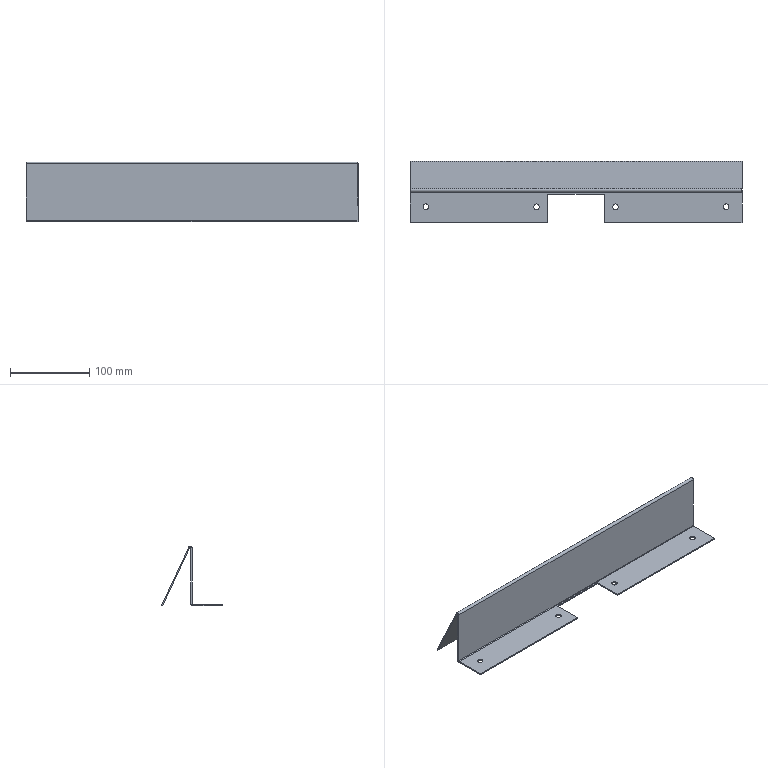Component | SolidWorks | Q1-A12-S21-Q4-05B-1 | 1 solid | 34 faces | box 420 x 77.3 x 75.36 mm | volume 119609 mm3 | plane 22 | cylinder 12 | commonest cylinder face diameters 7 x8 4.473 x2 1.473 x2 | material SUS-304
STEP:
#1=COLOUR_RGB('',0.7922,0.8196,0.9333);
#2=FILL_AREA_STYLE_COLOUR('',#1);
#3=FILL_AREA_STYLE('',(#2));
#4=SURFACE_STYLE_FILL_AREA(#3);
#5=SURFACE_SIDE_STYLE('',(#4));
#6=SURFACE_STYLE_USAGE(.BOTH.,#5);
#7=PRESENTATION_STYLE_ASSIGNMENT((#6));
#8=CARTESIAN_POINT('',(31.181,-0.7874,5.906));
#9=VERTEX_POINT('',#8);
#10=CARTESIAN_POINT('',(30.906,-0.7874,5.906));
#11=VERTEX_POINT('',#10);
#12=CARTESIAN_POINT('',(31.043,-0.7874,5.906));
#13=DIRECTION('',(0.,0.,-1.));
#14=DIRECTION('',(-1.,0.,0.));
#15=AXIS2_PLACEMENT_3D('',#12,#13,#14);
#16=CIRCLE('',#15,0.1378);
#17=EDGE_CURVE('',#9,#11,#16,.T.);
#18=ORIENTED_EDGE('',*,*,#17,.T.);
#19=CARTESIAN_POINT('',(30.906,-0.7874,5.965));
#20=VERTEX_POINT('',#19);
#21=CARTESIAN_POINT('',(30.906,-0.7874,5.965));
#22=DIRECTION('',(0.,0.,1.));
#23=VECTOR('',#22,39.37);
#24=LINE('',#21,#23);
#25=EDGE_CURVE('',#11,#20,#24,.T.);
#26=ORIENTED_EDGE('',*,*,#25,.T.);
#27=CARTESIAN_POINT('',(31.181,-0.7874,5.965));
#28=VERTEX_POINT('',#27);
#29=CARTESIAN_POINT('',(31.043,-0.7874,5.965));
#30=DIRECTION('',(0.,0.,1.));
#31=DIRECTION('',(1.,0.,0.));
#32=AXIS2_PLACEMENT_3D('',#29,#30,#31);
#33=CIRCLE('',#32,0.1378);
#34=EDGE_CURVE('',#20,#28,#33,.T.);
#35=ORIENTED_EDGE('',*,*,#34,.T.);
#36=CARTESIAN_POINT('',(31.181,-0.7874,5.965));
#37=DIRECTION('',(0.,0.,1.));
#38=VECTOR('',#37,39.37);
#39=LINE('',#36,#38);
#40=EDGE_CURVE('',#9,#28,#39,.T.);
#41=ORIENTED_EDGE('',*,*,#40,.F.);
#42=EDGE_LOOP('',(#18,#26,#35,#41));
#43=FACE_OUTER_BOUND('',#42,.T.);
#44=CARTESIAN_POINT('',(31.043,-0.7874,5.965));
#45=DIRECTION('',(0.,0.,1.));
#46=DIRECTION('',(1.,0.,0.));
#47=AXIS2_PLACEMENT_3D('',#44,#45,#46);
#48=CYLINDRICAL_SURFACE('',#47,0.1378);
#49=ADVANCED_FACE('',(#43),#48,.F.);
#50=CARTESIAN_POINT('',(25.669,-0.7874,5.906));
#51=VERTEX_POINT('',#50);
#52=CARTESIAN_POINT('',(25.394,-0.7874,5.906));
#53=VERTEX_POINT('',#52);
#54=CARTESIAN_POINT('',(25.531,-0.7874,5.906));
#55=DIRECTION('',(0.,0.,-1.));
#56=DIRECTION('',(-1.,0.,0.));
#57=AXIS2_PLACEMENT_3D('',#54,#55,#56);
#58=CIRCLE('',#57,0.1378);
#59=EDGE_CURVE('',#51,#53,#58,.T.);
#60=ORIENTED_EDGE('',*,*,#59,.T.);
#61=CARTESIAN_POINT('',(25.394,-0.7874,5.965));
#62=VERTEX_POINT('',#61);
#63=CARTESIAN_POINT('',(25.394,-0.7874,5.965));
#64=DIRECTION('',(0.,0.,1.));
#65=VECTOR('',#64,39.37);
#66=LINE('',#63,#65);
#67=EDGE_CURVE('',#53,#62,#66,.T.);
#68=ORIENTED_EDGE('',*,*,#67,.T.);
#69=CARTESIAN_POINT('',(25.669,-0.7874,5.965));
#70=VERTEX_POINT('',#69);
#71=CARTESIAN_POINT('',(25.531,-0.7874,5.965));
#72=DIRECTION('',(0.,0.,1.));
#73=DIRECTION('',(1.,0.,0.));
#74=AXIS2_PLACEMENT_3D('',#71,#72,#73);
#75=CIRCLE('',#74,0.1378);
#76=EDGE_CURVE('',#62,#70,#75,.T.);
#77=ORIENTED_EDGE('',*,*,#76,.T.);
#78=CARTESIAN_POINT('',(25.669,-0.7874,5.965));
#79=DIRECTION('',(0.,0.,1.));
#80=VECTOR('',#79,39.37);
#81=LINE('',#78,#80);
#82=EDGE_CURVE('',#51,#70,#81,.T.);
#83=ORIENTED_EDGE('',*,*,#82,.F.);
#84=EDGE_LOOP('',(#60,#68,#77,#83));
#85=FACE_OUTER_BOUND('',#84,.T.);
#86=CARTESIAN_POINT('',(25.531,-0.7874,5.965));
#87=DIRECTION('',(0.,0.,1.));
#88=DIRECTION('',(1.,0.,0.));
#89=AXIS2_PLACEMENT_3D('',#86,#87,#88);
#90=CYLINDRICAL_SURFACE('',#89,0.1378);
#91=ADVANCED_FACE('',(#85),#90,.F.);
#92=CARTESIAN_POINT('',(21.732,-0.7874,5.906));
#93=VERTEX_POINT('',#92);
#94=CARTESIAN_POINT('',(21.457,-0.7874,5.906));
#95=VERTEX_POINT('',#94);
#96=CARTESIAN_POINT('',(21.594,-0.7874,5.906));
#97=DIRECTION('',(0.,0.,-1.));
#98=DIRECTION('',(-1.,0.,0.));
#99=AXIS2_PLACEMENT_3D('',#96,#97,#98);
#100=CIRCLE('',#99,0.1378);
#101=EDGE_CURVE('',#93,#95,#100,.T.);
#102=ORIENTED_EDGE('',*,*,#101,.T.);
#103=CARTESIAN_POINT('',(21.457,-0.7874,5.965));
#104=VERTEX_POINT('',#103);
#105=CARTESIAN_POINT('',(21.457,-0.7874,5.965));
#106=DIRECTION('',(0.,0.,1.));
#107=VECTOR('',#106,39.37);
#108=LINE('',#105,#107);
#109=EDGE_CURVE('',#95,#104,#108,.T.);
#110=ORIENTED_EDGE('',*,*,#109,.T.);
#111=CARTESIAN_POINT('',(21.732,-0.7874,5.965));
#112=VERTEX_POINT('',#111);
#113=CARTESIAN_POINT('',(21.594,-0.7874,5.965));
#114=DIRECTION('',(0.,0.,1.));
#115=DIRECTION('',(1.,0.,0.));
#116=AXIS2_PLACEMENT_3D('',#113,#114,#115);
#117=CIRCLE('',#116,0.1378);
#118=EDGE_CURVE('',#104,#112,#117,.T.);
#119=ORIENTED_EDGE('',*,*,#118,.T.);
#120=CARTESIAN_POINT('',(21.732,-0.7874,5.965));
#121=DIRECTION('',(0.,0.,1.));
#122=VECTOR('',#121,39.37);
#123=LINE('',#120,#122);
#124=EDGE_CURVE('',#93,#112,#123,.T.);
#125=ORIENTED_EDGE('',*,*,#124,.F.);
#126=EDGE_LOOP('',(#102,#110,#119,#125));
#127=FACE_OUTER_BOUND('',#126,.T.);
#128=CARTESIAN_POINT('',(21.594,-0.7874,5.965));
#129=DIRECTION('',(0.,0.,1.));
#130=DIRECTION('',(1.,0.,0.));
#131=AXIS2_PLACEMENT_3D('',#128,#129,#130);
#132=CYLINDRICAL_SURFACE('',#131,0.1378);
#133=ADVANCED_FACE('',(#127),#132,.F.);
#134=CARTESIAN_POINT('',(16.22,-0.7874,5.906));
#135=VERTEX_POINT('',#134);
#136=CARTESIAN_POINT('',(15.945,-0.7874,5.906));
#137=VERTEX_POINT('',#136);
#138=CARTESIAN_POINT('',(16.083,-0.7874,5.906));
#139=DIRECTION('',(0.,0.,-1.));
#140=DIRECTION('',(-1.,0.,0.));
#141=AXIS2_PLACEMENT_3D('',#138,#139,#140);
#142=CIRCLE('',#141,0.1378);
#143=EDGE_CURVE('',#135,#137,#142,.T.);
#144=ORIENTED_EDGE('',*,*,#143,.T.);
#145=CARTESIAN_POINT('',(15.945,-0.7874,5.965));
#146=VERTEX_POINT('',#145);
#147=CARTESIAN_POINT('',(15.945,-0.7874,5.965));
#148=DIRECTION('',(0.,0.,1.));
#149=VECTOR('',#148,39.37);
#150=LINE('',#147,#149);
#151=EDGE_CURVE('',#137,#146,#150,.T.);
#152=ORIENTED_EDGE('',*,*,#151,.T.);
#153=CARTESIAN_POINT('',(16.22,-0.7874,5.965));
#154=VERTEX_POINT('',#153);
#155=CARTESIAN_POINT('',(16.083,-0.7874,5.965));
#156=DIRECTION('',(0.,0.,1.));
#157=DIRECTION('',(1.,0.,0.));
#158=AXIS2_PLACEMENT_3D('',#155,#156,#157);
#159=CIRCLE('',#158,0.1378);
#160=EDGE_CURVE('',#146,#154,#159,.T.);
#161=ORIENTED_EDGE('',*,*,#160,.T.);
#162=CARTESIAN_POINT('',(16.22,-0.7874,5.965));
#163=DIRECTION('',(0.,0.,1.));
#164=VECTOR('',#163,39.37);
#165=LINE('',#162,#164);
#166=EDGE_CURVE('',#135,#154,#165,.T.);
#167=ORIENTED_EDGE('',*,*,#166,.F.);
#168=EDGE_LOOP('',(#144,#152,#161,#167));
#169=FACE_OUTER_BOUND('',#168,.T.);
#170=CARTESIAN_POINT('',(16.083,-0.7874,5.965));
#171=DIRECTION('',(0.,0.,1.));
#172=DIRECTION('',(1.,0.,0.));
#173=AXIS2_PLACEMENT_3D('',#170,#171,#172);
#174=CYLINDRICAL_SURFACE('',#173,0.1378);
#175=ADVANCED_FACE('',(#169),#174,.F.);
#176=CARTESIAN_POINT('',(31.831,0.05528,8.797));
#177=VERTEX_POINT('',#176);
#178=CARTESIAN_POINT('',(31.831,1.404,5.906));
#179=VERTEX_POINT('',#178);
#180=CARTESIAN_POINT('',(31.831,1.518,5.66));
#181=DIRECTION('',(0.,0.4226,-0.9063));
#182=VECTOR('',#181,39.37);
#183=LINE('',#180,#182);
#184=EDGE_CURVE('',#177,#179,#183,.T.);
#185=ORIENTED_EDGE('',*,*,#184,.T.);
#186=CARTESIAN_POINT('',(31.831,1.469,5.906));
#187=VERTEX_POINT('',#186);
#188=CARTESIAN_POINT('',(31.831,1.572,5.906));
#189=DIRECTION('',(0.,1.,0.));
#190=VECTOR('',#189,39.37);
#191=LINE('',#188,#190);
#192=EDGE_CURVE('',#179,#187,#191,.T.);
#193=ORIENTED_EDGE('',*,*,#192,.T.);
#194=CARTESIAN_POINT('',(31.831,0.1088,8.822));
#195=VERTEX_POINT('',#194);
#196=CARTESIAN_POINT('',(31.831,1.097,6.703));
#197=DIRECTION('',(0.,0.4226,-0.9063));
#198=VECTOR('',#197,39.37);
#199=LINE('',#196,#198);
#200=EDGE_CURVE('',#195,#187,#199,.T.);
#201=ORIENTED_EDGE('',*,*,#200,.F.);
#202=CARTESIAN_POINT('',(31.831,0.05528,8.797));
#203=DIRECTION('',(0.,0.9063,0.4226));
#204=VECTOR('',#203,39.37);
#205=LINE('',#202,#204);
#206=EDGE_CURVE('',#177,#195,#205,.T.);
#207=ORIENTED_EDGE('',*,*,#206,.F.);
#208=EDGE_LOOP('',(#185,#193,#201,#207));
#209=FACE_OUTER_BOUND('',#208,.T.);
#210=CARTESIAN_POINT('',(31.831,1.572,5.685));
#211=DIRECTION('',(-1.,0.,0.));
#212=DIRECTION('',(0.,0.,1.));
#213=AXIS2_PLACEMENT_3D('',#210,#211,#212);
#214=PLANE('',#213);
#215=ADVANCED_FACE('',(#209),#214,.F.);
#216=CARTESIAN_POINT('',(15.295,1.469,5.906));
#217=VERTEX_POINT('',#216);
#218=CARTESIAN_POINT('',(15.295,0.1088,8.822));
#219=VERTEX_POINT('',#218);
#220=CARTESIAN_POINT('',(15.295,1.097,6.703));
#221=DIRECTION('',(0.,-0.4226,0.9063));
#222=VECTOR('',#221,39.37);
#223=LINE('',#220,#222);
#224=EDGE_CURVE('',#217,#219,#223,.T.);
#225=ORIENTED_EDGE('',*,*,#224,.F.);
#226=CARTESIAN_POINT('',(15.295,1.404,5.906));
#227=VERTEX_POINT('',#226);
#228=CARTESIAN_POINT('',(15.295,0.05352,5.906));
#229=DIRECTION('',(0.,-1.,0.));
#230=VECTOR('',#229,39.37);
#231=LINE('',#228,#230);
#232=EDGE_CURVE('',#217,#227,#231,.T.);
#233=ORIENTED_EDGE('',*,*,#232,.T.);
#234=CARTESIAN_POINT('',(15.295,0.05528,8.797));
#235=VERTEX_POINT('',#234);
#236=CARTESIAN_POINT('',(15.295,0.,8.915));
#237=DIRECTION('',(0.,-0.4226,0.9063));
#238=VECTOR('',#237,39.37);
#239=LINE('',#236,#238);
#240=EDGE_CURVE('',#227,#235,#239,.T.);
#241=ORIENTED_EDGE('',*,*,#240,.T.);
#242=CARTESIAN_POINT('',(15.295,0.1088,8.822));
#243=DIRECTION('',(0.,0.9063,0.4226));
#244=VECTOR('',#243,39.37);
#245=LINE('',#242,#244);
#246=EDGE_CURVE('',#235,#219,#245,.T.);
#247=ORIENTED_EDGE('',*,*,#246,.T.);
#248=EDGE_LOOP('',(#225,#233,#241,#247));
#249=FACE_OUTER_BOUND('',#248,.T.);
#250=CARTESIAN_POINT('',(15.295,0.05352,8.94));
#251=DIRECTION('',(1.,0.,0.));
#252=DIRECTION('',(0.,0.,-1.));
#253=AXIS2_PLACEMENT_3D('',#250,#251,#252);
#254=PLANE('',#253);
#255=ADVANCED_FACE('',(#249),#254,.F.);
#256=ORIENTED_EDGE('',*,*,#200,.T.);
#257=CARTESIAN_POINT('',(23.563,1.469,5.906));
#258=DIRECTION('',(-1.,0.,0.));
#259=VECTOR('',#258,39.37);
#260=LINE('',#257,#259);
#261=EDGE_CURVE('',#187,#217,#260,.T.);
#262=ORIENTED_EDGE('',*,*,#261,.T.);
#263=ORIENTED_EDGE('',*,*,#224,.T.);
#264=CARTESIAN_POINT('',(15.295,0.1088,8.822));
#265=DIRECTION('',(-1.,0.,-0.));
#266=VECTOR('',#265,39.37);
#267=LINE('',#264,#266);
#268=EDGE_CURVE('',#195,#219,#267,.T.);
#269=ORIENTED_EDGE('',*,*,#268,.F.);
#270=EDGE_LOOP('',(#256,#262,#263,#269));
#271=FACE_OUTER_BOUND('',#270,.T.);
#272=CARTESIAN_POINT('',(23.563,1.097,6.703));
#273=DIRECTION('',(0.,-0.9063,-0.4226));
#274=DIRECTION('',(0.,0.4226,-0.9063));
#275=AXIS2_PLACEMENT_3D('',#272,#273,#274);
#276=PLANE('',#275);
#277=ADVANCED_FACE('',(#271),#276,.F.);
#278=CARTESIAN_POINT('',(23.563,1.404,5.906));
#279=DIRECTION('',(-1.,0.,0.));
#280=VECTOR('',#279,39.37);
#281=LINE('',#278,#280);
#282=EDGE_CURVE('',#179,#227,#281,.T.);
#283=ORIENTED_EDGE('',*,*,#282,.F.);
#284=ORIENTED_EDGE('',*,*,#184,.F.);
#285=CARTESIAN_POINT('',(15.295,0.05528,8.797));
#286=DIRECTION('',(1.,-0.,0.));
#287=VECTOR('',#286,39.37);
#288=LINE('',#285,#287);
#289=EDGE_CURVE('',#235,#177,#288,.T.);
#290=ORIENTED_EDGE('',*,*,#289,.F.);
#291=ORIENTED_EDGE('',*,*,#240,.F.);
#292=EDGE_LOOP('',(#283,#284,#290,#291));
#293=FACE_OUTER_BOUND('',#292,.T.);
#294=CARTESIAN_POINT('',(23.563,1.043,6.678));
#295=DIRECTION('',(0.,-0.9063,-0.4226));
#296=DIRECTION('',(0.,0.4226,-0.9063));
#297=AXIS2_PLACEMENT_3D('',#294,#295,#296);
#298=PLANE('',#297);
#299=ADVANCED_FACE('',(#293),#298,.T.);
#300=CARTESIAN_POINT('',(22.146,-1.575,5.965));
#301=VERTEX_POINT('',#300);
#302=CARTESIAN_POINT('',(22.146,-1.575,5.906));
#303=VERTEX_POINT('',#302);
#304=CARTESIAN_POINT('',(22.146,-1.575,5.906));
#305=DIRECTION('',(0.,0.,-1.));
#306=VECTOR('',#305,39.37);
#307=LINE('',#304,#306);
#308=EDGE_CURVE('',#301,#303,#307,.T.);
#309=ORIENTED_EDGE('',*,*,#308,.F.);
#310=CARTESIAN_POINT('',(15.295,-1.575,5.965));
#311=VERTEX_POINT('',#310);
#312=CARTESIAN_POINT('',(15.295,-1.575,5.965));
#313=DIRECTION('',(1.,0.,0.));
#314=VECTOR('',#313,39.37);
#315=LINE('',#312,#314);
#316=EDGE_CURVE('',#311,#301,#315,.T.);
#317=ORIENTED_EDGE('',*,*,#316,.F.);
#318=CARTESIAN_POINT('',(15.295,-1.575,5.906));
#319=VERTEX_POINT('',#318);
#320=CARTESIAN_POINT('',(15.295,-1.575,5.906));
#321=DIRECTION('',(0.,0.,1.));
#322=VECTOR('',#321,39.37);
#323=LINE('',#320,#322);
#324=EDGE_CURVE('',#319,#311,#323,.T.);
#325=ORIENTED_EDGE('',*,*,#324,.F.);
#326=CARTESIAN_POINT('',(15.295,-1.575,5.906));
#327=DIRECTION('',(1.,0.,0.));
#328=VECTOR('',#327,39.37);
#329=LINE('',#326,#328);
#330=EDGE_CURVE('',#319,#303,#329,.T.);
#331=ORIENTED_EDGE('',*,*,#330,.T.);
#332=EDGE_LOOP('',(#309,#317,#325,#331));
#333=FACE_OUTER_BOUND('',#332,.T.);
#334=CARTESIAN_POINT('',(15.295,-1.575,5.906));
#335=DIRECTION('',(0.,-1.,0.));
#336=DIRECTION('',(0.,0.,-1.));
#337=AXIS2_PLACEMENT_3D('',#334,#335,#336);
#338=PLANE('',#337);
#339=ADVANCED_FACE('',(#333),#338,.T.);
#340=CARTESIAN_POINT('',(15.295,0.,8.785));
#341=VERTEX_POINT('',#340);
#342=CARTESIAN_POINT('',(15.295,-0.05906,8.785));
#343=VERTEX_POINT('',#342);
#344=CARTESIAN_POINT('',(15.295,0.,8.785));
#345=DIRECTION('',(0.,-1.,0.));
#346=VECTOR('',#345,39.37);
#347=LINE('',#344,#346);
#348=EDGE_CURVE('',#341,#343,#347,.T.);
#349=ORIENTED_EDGE('',*,*,#348,.F.);
#350=CARTESIAN_POINT('',(15.295,-0.,5.994));
#351=VERTEX_POINT('',#350);
#352=CARTESIAN_POINT('',(15.295,-0.,5.965));
#353=DIRECTION('',(-0.,0.,1.));
#354=VECTOR('',#353,39.37);
#355=LINE('',#352,#354);
#356=EDGE_CURVE('',#351,#341,#355,.T.);
#357=ORIENTED_EDGE('',*,*,#356,.F.);
#358=CARTESIAN_POINT('',(15.295,-0.05906,5.994));
#359=VERTEX_POINT('',#358);
#360=CARTESIAN_POINT('',(15.295,-0.05906,5.994));
#361=DIRECTION('',(0.,1.,-0.));
#362=VECTOR('',#361,39.37);
#363=LINE('',#360,#362);
#364=EDGE_CURVE('',#359,#351,#363,.T.);
#365=ORIENTED_EDGE('',*,*,#364,.F.);
#366=CARTESIAN_POINT('',(15.295,-0.05906,9.055));
#367=DIRECTION('',(-0.,0.,1.));
#368=VECTOR('',#367,39.37);
#369=LINE('',#366,#368);
#370=EDGE_CURVE('',#359,#343,#369,.T.);
#371=ORIENTED_EDGE('',*,*,#370,.T.);
#372=EDGE_LOOP('',(#349,#357,#365,#371));
#373=FACE_OUTER_BOUND('',#372,.T.);
#374=CARTESIAN_POINT('',(15.295,0.,9.055));
#375=DIRECTION('',(1.,0.,0.));
#376=DIRECTION('',(0.,0.,-1.));
#377=AXIS2_PLACEMENT_3D('',#374,#375,#376);
#378=PLANE('',#377);
#379=ADVANCED_FACE('',(#373),#378,.F.);
#380=CARTESIAN_POINT('',(31.831,0.,8.785));
#381=VERTEX_POINT('',#380);
#382=CARTESIAN_POINT('',(31.831,-0.05906,8.785));
#383=VERTEX_POINT('',#382);
#384=CARTESIAN_POINT('',(31.831,0.,8.785));
#385=DIRECTION('',(0.,-1.,0.));
#386=VECTOR('',#385,39.37);
#387=LINE('',#384,#386);
#388=EDGE_CURVE('',#381,#383,#387,.T.);
#389=ORIENTED_EDGE('',*,*,#388,.T.);
#390=CARTESIAN_POINT('',(31.831,-0.05906,5.994));
#391=VERTEX_POINT('',#390);
#392=CARTESIAN_POINT('',(31.831,-0.05906,5.965));
#393=DIRECTION('',(0.,-0.,-1.));
#394=VECTOR('',#393,39.37);
#395=LINE('',#392,#394);
#396=EDGE_CURVE('',#383,#391,#395,.T.);
#397=ORIENTED_EDGE('',*,*,#396,.T.);
#398=CARTESIAN_POINT('',(31.831,-0.,5.994));
#399=VERTEX_POINT('',#398);
#400=CARTESIAN_POINT('',(31.831,-0.,5.994));
#401=DIRECTION('',(0.,1.,-0.));
#402=VECTOR('',#401,39.37);
#403=LINE('',#400,#402);
#404=EDGE_CURVE('',#391,#399,#403,.T.);
#405=ORIENTED_EDGE('',*,*,#404,.T.);
#406=CARTESIAN_POINT('',(31.831,-0.,5.965));
#407=DIRECTION('',(0.,-0.,-1.));
#408=VECTOR('',#407,39.37);
#409=LINE('',#406,#408);
#410=EDGE_CURVE('',#381,#399,#409,.T.);
#411=ORIENTED_EDGE('',*,*,#410,.F.);
#412=EDGE_LOOP('',(#389,#397,#405,#411));
#413=FACE_OUTER_BOUND('',#412,.T.);
#414=CARTESIAN_POINT('',(31.831,-0.,5.965));
#415=DIRECTION('',(-1.,-0.,-0.));
#416=DIRECTION('',(-0.,0.,1.));
#417=AXIS2_PLACEMENT_3D('',#414,#415,#416);
#418=PLANE('',#417);
#419=ADVANCED_FACE('',(#413),#418,.F.);
#420=CARTESIAN_POINT('',(31.831,0.,8.785));
#421=DIRECTION('',(-1.,0.,0.));
#422=VECTOR('',#421,39.37);
#423=LINE('',#420,#422);
#424=EDGE_CURVE('',#381,#341,#423,.T.);
#425=ORIENTED_EDGE('',*,*,#424,.F.);
#426=ORIENTED_EDGE('',*,*,#410,.T.);
#427=CARTESIAN_POINT('',(31.831,-0.,5.994));
#428=DIRECTION('',(1.,-0.,-0.));
#429=VECTOR('',#428,39.37);
#430=LINE('',#427,#429);
#431=EDGE_CURVE('',#351,#399,#430,.T.);
#432=ORIENTED_EDGE('',*,*,#431,.F.);
#433=ORIENTED_EDGE('',*,*,#356,.T.);
#434=EDGE_LOOP('',(#425,#426,#432,#433));
#435=FACE_OUTER_BOUND('',#434,.T.);
#436=CARTESIAN_POINT('',(23.563,-0.,5.965));
#437=DIRECTION('',(0.,-1.,0.));
#438=DIRECTION('',(0.,-0.,-1.));
#439=AXIS2_PLACEMENT_3D('',#436,#437,#438);
#440=PLANE('',#439);
#441=ADVANCED_FACE('',(#435),#440,.F.);
#442=ORIENTED_EDGE('',*,*,#396,.F.);
#443=CARTESIAN_POINT('',(31.831,-0.05906,8.785));
#444=DIRECTION('',(-1.,0.,0.));
#445=VECTOR('',#444,39.37);
#446=LINE('',#443,#445);
#447=EDGE_CURVE('',#383,#343,#446,.T.);
#448=ORIENTED_EDGE('',*,*,#447,.T.);
#449=ORIENTED_EDGE('',*,*,#370,.F.);
#450=CARTESIAN_POINT('',(31.831,-0.05906,5.994));
#451=DIRECTION('',(-1.,0.,0.));
#452=VECTOR('',#451,39.37);
#453=LINE('',#450,#452);
#454=EDGE_CURVE('',#391,#359,#453,.T.);
#455=ORIENTED_EDGE('',*,*,#454,.F.);
#456=EDGE_LOOP('',(#442,#448,#449,#455));
#457=FACE_OUTER_BOUND('',#456,.T.);
#458=CARTESIAN_POINT('',(23.563,-0.05906,5.965));
#459=DIRECTION('',(0.,-1.,0.));
#460=DIRECTION('',(0.,-0.,-1.));
#461=AXIS2_PLACEMENT_3D('',#458,#459,#460);
#462=PLANE('',#461);
#463=ADVANCED_FACE('',(#457),#462,.T.);
#464=CARTESIAN_POINT('',(15.295,-0.08806,5.965));
#465=VERTEX_POINT('',#464);
#466=CARTESIAN_POINT('',(15.295,-1.575,5.965));
#467=DIRECTION('',(0.,-1.,0.));
#468=VECTOR('',#467,39.37);
#469=LINE('',#466,#468);
#470=EDGE_CURVE('',#465,#311,#469,.T.);
#471=ORIENTED_EDGE('',*,*,#470,.F.);
#472=CARTESIAN_POINT('',(15.295,-0.08806,5.906));
#473=VERTEX_POINT('',#472);
#474=CARTESIAN_POINT('',(15.295,-0.08806,5.965));
#475=DIRECTION('',(0.,0.,-1.));
#476=VECTOR('',#475,39.37);
#477=LINE('',#474,#476);
#478=EDGE_CURVE('',#465,#473,#477,.T.);
#479=ORIENTED_EDGE('',*,*,#478,.T.);
#480=CARTESIAN_POINT('',(15.295,-1.575,5.906));
#481=DIRECTION('',(0.,-1.,0.));
#482=VECTOR('',#481,39.37);
#483=LINE('',#480,#482);
#484=EDGE_CURVE('',#473,#319,#483,.T.);
#485=ORIENTED_EDGE('',*,*,#484,.T.);
#486=ORIENTED_EDGE('',*,*,#324,.T.);
#487=EDGE_LOOP('',(#471,#479,#485,#486));
#488=FACE_OUTER_BOUND('',#487,.T.);
#489=CARTESIAN_POINT('',(15.295,-1.575,5.906));
#490=DIRECTION('',(-1.,0.,0.));
#491=DIRECTION('',(0.,0.,1.));
#492=AXIS2_PLACEMENT_3D('',#489,#490,#491);
#493=PLANE('',#492);
#494=ADVANCED_FACE('',(#488),#493,.T.);
#495=ORIENTED_EDGE('',*,*,#17,.F.);
#496=CARTESIAN_POINT('',(31.043,-0.7874,5.906));
#497=DIRECTION('',(0.,0.,-1.));
#498=DIRECTION('',(-1.,0.,0.));
#499=AXIS2_PLACEMENT_3D('',#496,#497,#498);
#500=CIRCLE('',#499,0.1378);
#501=EDGE_CURVE('',#11,#9,#500,.T.);
#502=ORIENTED_EDGE('',*,*,#501,.F.);
#503=EDGE_LOOP('',(#495,#502));
#504=FACE_BOUND('',#503,.T.);
#505=ORIENTED_EDGE('',*,*,#59,.F.);
#506=CARTESIAN_POINT('',(25.531,-0.7874,5.906));
#507=DIRECTION('',(0.,0.,-1.));
#508=DIRECTION('',(-1.,0.,0.));
#509=AXIS2_PLACEMENT_3D('',#506,#507,#508);
#510=CIRCLE('',#509,0.1378);
#511=EDGE_CURVE('',#53,#51,#510,.T.);
#512=ORIENTED_EDGE('',*,*,#511,.F.);
#513=EDGE_LOOP('',(#505,#512));
#514=FACE_BOUND('',#513,.T.);
#515=ORIENTED_EDGE('',*,*,#101,.F.);
#516=CARTESIAN_POINT('',(21.594,-0.7874,5.906));
#517=DIRECTION('',(0.,0.,-1.));
#518=DIRECTION('',(-1.,0.,0.));
#519=AXIS2_PLACEMENT_3D('',#516,#517,#518);
#520=CIRCLE('',#519,0.1378);
#521=EDGE_CURVE('',#95,#93,#520,.T.);
#522=ORIENTED_EDGE('',*,*,#521,.F.);
#523=EDGE_LOOP('',(#515,#522));
#524=FACE_BOUND('',#523,.T.);
#525=ORIENTED_EDGE('',*,*,#143,.F.);
#526=CARTESIAN_POINT('',(16.083,-0.7874,5.906));
#527=DIRECTION('',(0.,0.,-1.));
#528=DIRECTION('',(-1.,0.,0.));
#529=AXIS2_PLACEMENT_3D('',#526,#527,#528);
#530=CIRCLE('',#529,0.1378);
#531=EDGE_CURVE('',#137,#135,#530,.T.);
#532=ORIENTED_EDGE('',*,*,#531,.F.);
#533=EDGE_LOOP('',(#525,#532));
#534=FACE_BOUND('',#533,.T.);
#535=CARTESIAN_POINT('',(22.146,-0.1575,5.906));
#536=VERTEX_POINT('',#535);
#537=CARTESIAN_POINT('',(22.146,-0.7874,5.906));
#538=DIRECTION('',(0.,1.,0.));
#539=VECTOR('',#538,39.37);
#540=LINE('',#537,#539);
#541=EDGE_CURVE('',#303,#536,#540,.T.);
#542=ORIENTED_EDGE('',*,*,#541,.F.);
#543=ORIENTED_EDGE('',*,*,#330,.F.);
#544=ORIENTED_EDGE('',*,*,#484,.F.);
#545=CARTESIAN_POINT('',(31.831,-0.08806,5.906));
#546=VERTEX_POINT('',#545);
#547=CARTESIAN_POINT('',(15.295,-0.08806,5.906));
#548=DIRECTION('',(1.,0.,0.));
#549=VECTOR('',#548,39.37);
#550=LINE('',#547,#549);
#551=EDGE_CURVE('',#473,#546,#550,.T.);
#552=ORIENTED_EDGE('',*,*,#551,.T.);
#553=CARTESIAN_POINT('',(31.831,-1.575,5.906));
#554=VERTEX_POINT('',#553);
#555=CARTESIAN_POINT('',(31.831,-1.575,5.906));
#556=DIRECTION('',(0.,1.,0.));
#557=VECTOR('',#556,39.37);
#558=LINE('',#555,#557);
#559=EDGE_CURVE('',#554,#546,#558,.T.);
#560=ORIENTED_EDGE('',*,*,#559,.F.);
#561=CARTESIAN_POINT('',(24.98,-1.575,5.906));
#562=VERTEX_POINT('',#561);
#563=CARTESIAN_POINT('',(15.295,-1.575,5.906));
#564=DIRECTION('',(1.,0.,0.));
#565=VECTOR('',#564,39.37);
#566=LINE('',#563,#565);
#567=EDGE_CURVE('',#562,#554,#566,.T.);
#568=ORIENTED_EDGE('',*,*,#567,.F.);
#569=CARTESIAN_POINT('',(24.98,-0.1575,5.906));
#570=VERTEX_POINT('',#569);
#571=CARTESIAN_POINT('',(24.98,-0.7874,5.906));
#572=DIRECTION('',(0.,-1.,0.));
#573=VECTOR('',#572,39.37);
#574=LINE('',#571,#573);
#575=EDGE_CURVE('',#570,#562,#574,.T.);
#576=ORIENTED_EDGE('',*,*,#575,.F.);
#577=CARTESIAN_POINT('',(23.563,-0.1575,5.906));
#578=DIRECTION('',(1.,0.,0.));
#579=VECTOR('',#578,39.37);
#580=LINE('',#577,#579);
#581=EDGE_CURVE('',#536,#570,#580,.T.);
#582=ORIENTED_EDGE('',*,*,#581,.F.);
#583=EDGE_LOOP('',(#542,#543,#544,#552,#560,#568,#576,#582));
#584=FACE_OUTER_BOUND('',#583,.T.);
#585=CARTESIAN_POINT('',(23.563,-0.7874,5.906));
#586=DIRECTION('',(0.,0.,-1.));
#587=DIRECTION('',(-1.,0.,0.));
#588=AXIS2_PLACEMENT_3D('',#585,#586,#587);
#589=PLANE('',#588);
#590=ADVANCED_FACE('',(#504,#514,#524,#534,#584),#589,.T.);
#591=CARTESIAN_POINT('',(31.043,-0.7874,5.965));
#592=DIRECTION('',(0.,0.,1.));
#593=DIRECTION('',(1.,0.,0.));
#594=AXIS2_PLACEMENT_3D('',#591,#592,#593);
#595=CIRCLE('',#594,0.1378);
#596=EDGE_CURVE('',#28,#20,#595,.T.);
#597=ORIENTED_EDGE('',*,*,#596,.F.);
#598=ORIENTED_EDGE('',*,*,#34,.F.);
#599=EDGE_LOOP('',(#597,#598));
#600=FACE_BOUND('',#599,.T.);
#601=CARTESIAN_POINT('',(25.531,-0.7874,5.965));
#602=DIRECTION('',(0.,0.,1.));
#603=DIRECTION('',(1.,0.,0.));
#604=AXIS2_PLACEMENT_3D('',#601,#602,#603);
#605=CIRCLE('',#604,0.1378);
#606=EDGE_CURVE('',#70,#62,#605,.T.);
#607=ORIENTED_EDGE('',*,*,#606,.F.);
#608=ORIENTED_EDGE('',*,*,#76,.F.);
#609=EDGE_LOOP('',(#607,#608));
#610=FACE_BOUND('',#609,.T.);
#611=CARTESIAN_POINT('',(21.594,-0.7874,5.965));
#612=DIRECTION('',(0.,0.,1.));
#613=DIRECTION('',(1.,0.,0.));
#614=AXIS2_PLACEMENT_3D('',#611,#612,#613);
#615=CIRCLE('',#614,0.1378);
#616=EDGE_CURVE('',#112,#104,#615,.T.);
#617=ORIENTED_EDGE('',*,*,#616,.F.);
#618=ORIENTED_EDGE('',*,*,#118,.F.);
#619=EDGE_LOOP('',(#617,#618));
#620=FACE_BOUND('',#619,.T.);
#621=CARTESIAN_POINT('',(16.083,-0.7874,5.965));
#622=DIRECTION('',(0.,0.,1.));
#623=DIRECTION('',(1.,0.,0.));
#624=AXIS2_PLACEMENT_3D('',#621,#622,#623);
#625=CIRCLE('',#624,0.1378);
#626=EDGE_CURVE('',#154,#146,#625,.T.);
#627=ORIENTED_EDGE('',*,*,#626,.F.);
#628=ORIENTED_EDGE('',*,*,#160,.F.);
#629=EDGE_LOOP('',(#627,#628));
#630=FACE_BOUND('',#629,.T.);
#631=ORIENTED_EDGE('',*,*,#316,.T.);
#632=CARTESIAN_POINT('',(22.146,-0.1575,5.965));
#633=VERTEX_POINT('',#632);
#634=CARTESIAN_POINT('',(22.146,-1.575,5.965));
#635=DIRECTION('',(0.,-1.,0.));
#636=VECTOR('',#635,39.37);
#637=LINE('',#634,#636);
#638=EDGE_CURVE('',#633,#301,#637,.T.);
#639=ORIENTED_EDGE('',*,*,#638,.F.);
#640=CARTESIAN_POINT('',(24.98,-0.1575,5.965));
#641=VERTEX_POINT('',#640);
#642=CARTESIAN_POINT('',(22.146,-0.1575,5.965));
#643=DIRECTION('',(-1.,0.,0.));
#644=VECTOR('',#643,39.37);
#645=LINE('',#642,#644);
#646=EDGE_CURVE('',#641,#633,#645,.T.);
#647=ORIENTED_EDGE('',*,*,#646,.F.);
#648=CARTESIAN_POINT('',(24.98,-1.575,5.965));
#649=VERTEX_POINT('',#648);
#650=CARTESIAN_POINT('',(24.98,-1.575,5.965));
#651=DIRECTION('',(0.,1.,0.));
#652=VECTOR('',#651,39.37);
#653=LINE('',#650,#652);
#654=EDGE_CURVE('',#649,#641,#653,.T.);
#655=ORIENTED_EDGE('',*,*,#654,.F.);
#656=CARTESIAN_POINT('',(31.831,-1.575,5.965));
#657=VERTEX_POINT('',#656);
#658=CARTESIAN_POINT('',(15.295,-1.575,5.965));
#659=DIRECTION('',(1.,0.,0.));
#660=VECTOR('',#659,39.37);
#661=LINE('',#658,#660);
#662=EDGE_CURVE('',#649,#657,#661,.T.);
#663=ORIENTED_EDGE('',*,*,#662,.T.);
#664=CARTESIAN_POINT('',(31.831,-0.08806,5.965));
#665=VERTEX_POINT('',#664);
#666=CARTESIAN_POINT('',(31.831,-1.575,5.965));
#667=DIRECTION('',(0.,1.,0.));
#668=VECTOR('',#667,39.37);
#669=LINE('',#666,#668);
#670=EDGE_CURVE('',#657,#665,#669,.T.);
#671=ORIENTED_EDGE('',*,*,#670,.T.);
#672=CARTESIAN_POINT('',(15.295,-0.08806,5.965));
#673=DIRECTION('',(1.,0.,0.));
#674=VECTOR('',#673,39.37);
#675=LINE('',#672,#674);
#676=EDGE_CURVE('',#465,#665,#675,.T.);
#677=ORIENTED_EDGE('',*,*,#676,.F.);
#678=ORIENTED_EDGE('',*,*,#470,.T.);
#679=EDGE_LOOP('',(#631,#639,#647,#655,#663,#671,#677,#678));
#680=FACE_OUTER_BOUND('',#679,.T.);
#681=CARTESIAN_POINT('',(23.563,-0.7874,5.965));
#682=DIRECTION('',(0.,0.,-1.));
#683=DIRECTION('',(-1.,0.,0.));
#684=AXIS2_PLACEMENT_3D('',#681,#682,#683);
#685=PLANE('',#684);
#686=ADVANCED_FACE('',(#600,#610,#620,#630,#680),#685,.F.);
#687=CARTESIAN_POINT('',(31.831,-0.08806,5.965));
#688=DIRECTION('',(0.,0.,-1.));
#689=VECTOR('',#688,39.37);
#690=LINE('',#687,#689);
#691=EDGE_CURVE('',#665,#546,#690,.T.);
#692=ORIENTED_EDGE('',*,*,#691,.F.);
#693=ORIENTED_EDGE('',*,*,#670,.F.);
#694=CARTESIAN_POINT('',(31.831,-1.575,5.906));
#695=DIRECTION('',(0.,0.,1.));
#696=VECTOR('',#695,39.37);
#697=LINE('',#694,#696);
#698=EDGE_CURVE('',#554,#657,#697,.T.);
#699=ORIENTED_EDGE('',*,*,#698,.F.);
#700=ORIENTED_EDGE('',*,*,#559,.T.);
#701=EDGE_LOOP('',(#692,#693,#699,#700));
#702=FACE_OUTER_BOUND('',#701,.T.);
#703=CARTESIAN_POINT('',(31.831,-1.575,5.906));
#704=DIRECTION('',(1.,0.,0.));
#705=DIRECTION('',(0.,0.,-1.));
#706=AXIS2_PLACEMENT_3D('',#703,#704,#705);
#707=PLANE('',#706);
#708=ADVANCED_FACE('',(#702),#707,.T.);
#709=CARTESIAN_POINT('',(24.98,-1.575,5.906));
#710=DIRECTION('',(0.,0.,1.));
#711=VECTOR('',#710,39.37);
#712=LINE('',#709,#711);
#713=EDGE_CURVE('',#562,#649,#712,.T.);
#714=ORIENTED_EDGE('',*,*,#713,.F.);
#715=ORIENTED_EDGE('',*,*,#567,.T.);
#716=ORIENTED_EDGE('',*,*,#698,.T.);
#717=ORIENTED_EDGE('',*,*,#662,.F.);
#718=EDGE_LOOP('',(#714,#715,#716,#717));
#719=FACE_OUTER_BOUND('',#718,.T.);
#720=CARTESIAN_POINT('',(15.295,-1.575,5.906));
#721=DIRECTION('',(0.,-1.,0.));
#722=DIRECTION('',(0.,0.,-1.));
#723=AXIS2_PLACEMENT_3D('',#720,#721,#722);
#724=PLANE('',#723);
#725=ADVANCED_FACE('',(#719),#724,.T.);
#726=ORIENTED_EDGE('',*,*,#404,.F.);
#727=CARTESIAN_POINT('',(31.831,-0.08806,5.994));
#728=DIRECTION('',(1.,0.,0.));
#729=DIRECTION('',(0.,0.,1.));
#730=AXIS2_PLACEMENT_3D('',#727,#728,#729);
#731=CIRCLE('',#730,0.029);
#732=EDGE_CURVE('',#665,#391,#731,.T.);
#733=ORIENTED_EDGE('',*,*,#732,.F.);
#734=ORIENTED_EDGE('',*,*,#691,.T.);
#735=CARTESIAN_POINT('',(31.831,-0.08806,5.994));
#736=DIRECTION('',(1.,0.,0.));
#737=DIRECTION('',(0.,0.,1.));
#738=AXIS2_PLACEMENT_3D('',#735,#736,#737);
#739=CIRCLE('',#738,0.08806);
#740=EDGE_CURVE('',#546,#399,#739,.T.);
#741=ORIENTED_EDGE('',*,*,#740,.T.);
#742=EDGE_LOOP('',(#726,#733,#734,#741));
#743=FACE_OUTER_BOUND('',#742,.T.);
#744=CARTESIAN_POINT('',(31.831,-0.08806,5.994));
#745=DIRECTION('',(1.,0.,0.));
#746=DIRECTION('',(0.,0.,-1.));
#747=AXIS2_PLACEMENT_3D('',#744,#745,#746);
#748=PLANE('',#747);
#749=ADVANCED_FACE('',(#743),#748,.T.);
#750=CARTESIAN_POINT('',(15.295,-0.08806,5.994));
#751=DIRECTION('',(-1.,0.,0.));
#752=DIRECTION('',(0.,0.,1.));
#753=AXIS2_PLACEMENT_3D('',#750,#751,#752);
#754=CIRCLE('',#753,0.029);
#755=EDGE_CURVE('',#359,#465,#754,.T.);
#756=ORIENTED_EDGE('',*,*,#755,.F.);
#757=ORIENTED_EDGE('',*,*,#364,.T.);
#758=CARTESIAN_POINT('',(15.295,-0.08806,5.994));
#759=DIRECTION('',(-1.,0.,0.));
#760=DIRECTION('',(0.,0.,1.));
#761=AXIS2_PLACEMENT_3D('',#758,#759,#760);
#762=CIRCLE('',#761,0.08806);
#763=EDGE_CURVE('',#351,#473,#762,.T.);
#764=ORIENTED_EDGE('',*,*,#763,.T.);
#765=ORIENTED_EDGE('',*,*,#478,.F.);
#766=EDGE_LOOP('',(#756,#757,#764,#765));
#767=FACE_OUTER_BOUND('',#766,.T.);
#768=CARTESIAN_POINT('',(15.295,-0.08806,5.994));
#769=DIRECTION('',(1.,0.,0.));
#770=DIRECTION('',(0.,0.,-1.));
#771=AXIS2_PLACEMENT_3D('',#768,#769,#770);
#772=PLANE('',#771);
#773=ADVANCED_FACE('',(#767),#772,.F.);
#774=ORIENTED_EDGE('',*,*,#551,.F.);
#775=ORIENTED_EDGE('',*,*,#763,.F.);
#776=ORIENTED_EDGE('',*,*,#431,.T.);
#777=ORIENTED_EDGE('',*,*,#740,.F.);
#778=EDGE_LOOP('',(#774,#775,#776,#777));
#779=FACE_OUTER_BOUND('',#778,.T.);
#780=CARTESIAN_POINT('',(15.295,-0.08806,5.994));
#781=DIRECTION('',(-1.,0.,0.));
#782=DIRECTION('',(0.,1.,0.));
#783=AXIS2_PLACEMENT_3D('',#780,#781,#782);
#784=CYLINDRICAL_SURFACE('',#783,0.08806);
#785=ADVANCED_FACE('',(#779),#784,.T.);
#786=ORIENTED_EDGE('',*,*,#676,.T.);
#787=ORIENTED_EDGE('',*,*,#732,.T.);
#788=ORIENTED_EDGE('',*,*,#454,.T.);
#789=ORIENTED_EDGE('',*,*,#755,.T.);
#790=EDGE_LOOP('',(#786,#787,#788,#789));
#791=FACE_OUTER_BOUND('',#790,.T.);
#792=CARTESIAN_POINT('',(15.295,-0.08806,5.994));
#793=DIRECTION('',(-1.,0.,0.));
#794=DIRECTION('',(0.,1.,0.));
#795=AXIS2_PLACEMENT_3D('',#792,#793,#794);
#796=CYLINDRICAL_SURFACE('',#795,0.029);
#797=ADVANCED_FACE('',(#791),#796,.F.);
#798=ORIENTED_EDGE('',*,*,#246,.F.);
#799=CARTESIAN_POINT('',(15.295,0.029,8.785));
#800=DIRECTION('',(-1.,0.,0.));
#801=DIRECTION('',(0.,-0.,-1.));
#802=AXIS2_PLACEMENT_3D('',#799,#800,#801);
#803=CIRCLE('',#802,0.029);
#804=EDGE_CURVE('',#341,#235,#803,.T.);
#805=ORIENTED_EDGE('',*,*,#804,.F.);
#806=ORIENTED_EDGE('',*,*,#348,.T.);
#807=CARTESIAN_POINT('',(15.295,0.029,8.785));
#808=DIRECTION('',(-1.,0.,0.));
#809=DIRECTION('',(0.,0.,-1.));
#810=AXIS2_PLACEMENT_3D('',#807,#808,#809);
#811=CIRCLE('',#810,0.08806);
#812=EDGE_CURVE('',#343,#219,#811,.T.);
#813=ORIENTED_EDGE('',*,*,#812,.T.);
#814=EDGE_LOOP('',(#798,#805,#806,#813));
#815=FACE_OUTER_BOUND('',#814,.T.);
#816=CARTESIAN_POINT('',(15.295,0.029,8.785));
#817=DIRECTION('',(-1.,0.,0.));
#818=DIRECTION('',(0.,0.,1.));
#819=AXIS2_PLACEMENT_3D('',#816,#817,#818);
#820=PLANE('',#819);
#821=ADVANCED_FACE('',(#815),#820,.T.);
#822=CARTESIAN_POINT('',(31.831,0.029,8.785));
#823=DIRECTION('',(1.,0.,0.));
#824=DIRECTION('',(0.,0.,-1.));
#825=AXIS2_PLACEMENT_3D('',#822,#823,#824);
#826=CIRCLE('',#825,0.029);
#827=EDGE_CURVE('',#177,#381,#826,.T.);
#828=ORIENTED_EDGE('',*,*,#827,.F.);
#829=ORIENTED_EDGE('',*,*,#206,.T.);
#830=CARTESIAN_POINT('',(31.831,0.029,8.785));
#831=DIRECTION('',(1.,0.,0.));
#832=DIRECTION('',(0.,0.,-1.));
#833=AXIS2_PLACEMENT_3D('',#830,#831,#832);
#834=CIRCLE('',#833,0.08806);
#835=EDGE_CURVE('',#195,#383,#834,.T.);
#836=ORIENTED_EDGE('',*,*,#835,.T.);
#837=ORIENTED_EDGE('',*,*,#388,.F.);
#838=EDGE_LOOP('',(#828,#829,#836,#837));
#839=FACE_OUTER_BOUND('',#838,.T.);
#840=CARTESIAN_POINT('',(31.831,0.029,8.785));
#841=DIRECTION('',(-1.,0.,0.));
#842=DIRECTION('',(0.,0.,1.));
#843=AXIS2_PLACEMENT_3D('',#840,#841,#842);
#844=PLANE('',#843);
#845=ADVANCED_FACE('',(#839),#844,.F.);
#846=ORIENTED_EDGE('',*,*,#447,.F.);
#847=ORIENTED_EDGE('',*,*,#835,.F.);
#848=ORIENTED_EDGE('',*,*,#268,.T.);
#849=ORIENTED_EDGE('',*,*,#812,.F.);
#850=EDGE_LOOP('',(#846,#847,#848,#849));
#851=FACE_OUTER_BOUND('',#850,.T.);
#852=CARTESIAN_POINT('',(31.831,0.029,8.785));
#853=DIRECTION('',(1.,0.,0.));
#854=DIRECTION('',(0.,0.9063,0.4226));
#855=AXIS2_PLACEMENT_3D('',#852,#853,#854);
#856=CYLINDRICAL_SURFACE('',#855,0.08806);
#857=ADVANCED_FACE('',(#851),#856,.T.);
#858=ORIENTED_EDGE('',*,*,#424,.T.);
#859=ORIENTED_EDGE('',*,*,#804,.T.);
#860=ORIENTED_EDGE('',*,*,#289,.T.);
#861=ORIENTED_EDGE('',*,*,#827,.T.);
#862=EDGE_LOOP('',(#858,#859,#860,#861));
#863=FACE_OUTER_BOUND('',#862,.T.);
#864=CARTESIAN_POINT('',(31.831,0.029,8.785));
#865=DIRECTION('',(1.,0.,0.));
#866=DIRECTION('',(0.,0.9063,0.4226));
#867=AXIS2_PLACEMENT_3D('',#864,#865,#866);
#868=CYLINDRICAL_SURFACE('',#867,0.029);
#869=ADVANCED_FACE('',(#863),#868,.F.);
#870=ORIENTED_EDGE('',*,*,#541,.T.);
#871=CARTESIAN_POINT('',(22.146,-0.1575,5.66));
#872=DIRECTION('',(0.,0.,1.));
#873=VECTOR('',#872,39.37);
#874=LINE('',#871,#873);
#875=EDGE_CURVE('',#536,#633,#874,.T.);
#876=ORIENTED_EDGE('',*,*,#875,.T.);
#877=ORIENTED_EDGE('',*,*,#638,.T.);
#878=ORIENTED_EDGE('',*,*,#308,.T.);
#879=EDGE_LOOP('',(#870,#876,#877,#878));
#880=FACE_OUTER_BOUND('',#879,.T.);
#881=CARTESIAN_POINT('',(22.146,-1.575,5.66));
#882=DIRECTION('',(-1.,0.,0.));
#883=DIRECTION('',(0.,0.,1.));
#884=AXIS2_PLACEMENT_3D('',#881,#882,#883);
#885=PLANE('',#884);
#886=ADVANCED_FACE('',(#880),#885,.F.);
#887=ORIENTED_EDGE('',*,*,#581,.T.);
#888=CARTESIAN_POINT('',(24.98,-0.1575,5.66));
#889=DIRECTION('',(0.,0.,1.));
#890=VECTOR('',#889,39.37);
#891=LINE('',#888,#890);
#892=EDGE_CURVE('',#570,#641,#891,.T.);
#893=ORIENTED_EDGE('',*,*,#892,.T.);
#894=ORIENTED_EDGE('',*,*,#646,.T.);
#895=ORIENTED_EDGE('',*,*,#875,.F.);
#896=EDGE_LOOP('',(#887,#893,#894,#895));
#897=FACE_OUTER_BOUND('',#896,.T.);
#898=CARTESIAN_POINT('',(22.146,-0.1575,5.66));
#899=DIRECTION('',(0.,1.,0.));
#900=DIRECTION('',(0.,0.,1.));
#901=AXIS2_PLACEMENT_3D('',#898,#899,#900);
#902=PLANE('',#901);
#903=ADVANCED_FACE('',(#897),#902,.F.);
#904=ORIENTED_EDGE('',*,*,#575,.T.);
#905=ORIENTED_EDGE('',*,*,#713,.T.);
#906=ORIENTED_EDGE('',*,*,#654,.T.);
#907=ORIENTED_EDGE('',*,*,#892,.F.);
#908=EDGE_LOOP('',(#904,#905,#906,#907));
#909=FACE_OUTER_BOUND('',#908,.T.);
#910=CARTESIAN_POINT('',(24.98,-1.575,5.66));
#911=DIRECTION('',(1.,0.,0.));
#912=DIRECTION('',(0.,0.,-1.));
#913=AXIS2_PLACEMENT_3D('',#910,#911,#912);
#914=PLANE('',#913);
#915=ADVANCED_FACE('',(#909),#914,.F.);
#916=ORIENTED_EDGE('',*,*,#151,.F.);
#917=ORIENTED_EDGE('',*,*,#531,.T.);
#918=ORIENTED_EDGE('',*,*,#166,.T.);
#919=ORIENTED_EDGE('',*,*,#626,.T.);
#920=EDGE_LOOP('',(#916,#917,#918,#919));
#921=FACE_OUTER_BOUND('',#920,.T.);
#922=CARTESIAN_POINT('',(16.083,-0.7874,5.965));
#923=DIRECTION('',(0.,0.,1.));
#924=DIRECTION('',(1.,0.,0.));
#925=AXIS2_PLACEMENT_3D('',#922,#923,#924);
#926=CYLINDRICAL_SURFACE('',#925,0.1378);
#927=ADVANCED_FACE('',(#921),#926,.F.);
#928=ORIENTED_EDGE('',*,*,#109,.F.);
#929=ORIENTED_EDGE('',*,*,#521,.T.);
#930=ORIENTED_EDGE('',*,*,#124,.T.);
#931=ORIENTED_EDGE('',*,*,#616,.T.);
#932=EDGE_LOOP('',(#928,#929,#930,#931));
#933=FACE_OUTER_BOUND('',#932,.T.);
#934=CARTESIAN_POINT('',(21.594,-0.7874,5.965));
#935=DIRECTION('',(0.,0.,1.));
#936=DIRECTION('',(1.,0.,0.));
#937=AXIS2_PLACEMENT_3D('',#934,#935,#936);
#938=CYLINDRICAL_SURFACE('',#937,0.1378);
#939=ADVANCED_FACE('',(#933),#938,.F.);
#940=ORIENTED_EDGE('',*,*,#67,.F.);
#941=ORIENTED_EDGE('',*,*,#511,.T.);
#942=ORIENTED_EDGE('',*,*,#82,.T.);
#943=ORIENTED_EDGE('',*,*,#606,.T.);
#944=EDGE_LOOP('',(#940,#941,#942,#943));
#945=FACE_OUTER_BOUND('',#944,.T.);
#946=CARTESIAN_POINT('',(25.531,-0.7874,5.965));
#947=DIRECTION('',(0.,0.,1.));
#948=DIRECTION('',(1.,0.,0.));
#949=AXIS2_PLACEMENT_3D('',#946,#947,#948);
#950=CYLINDRICAL_SURFACE('',#949,0.1378);
#951=ADVANCED_FACE('',(#945),#950,.F.);
#952=ORIENTED_EDGE('',*,*,#25,.F.);
#953=ORIENTED_EDGE('',*,*,#501,.T.);
#954=ORIENTED_EDGE('',*,*,#40,.T.);
#955=ORIENTED_EDGE('',*,*,#596,.T.);
#956=EDGE_LOOP('',(#952,#953,#954,#955));
#957=FACE_OUTER_BOUND('',#956,.T.);
#958=CARTESIAN_POINT('',(31.043,-0.7874,5.965));
#959=DIRECTION('',(0.,0.,1.));
#960=DIRECTION('',(1.,0.,0.));
#961=AXIS2_PLACEMENT_3D('',#958,#959,#960);
#962=CYLINDRICAL_SURFACE('',#961,0.1378);
#963=ADVANCED_FACE('',(#957),#962,.F.);
#964=ORIENTED_EDGE('',*,*,#192,.F.);
#965=ORIENTED_EDGE('',*,*,#282,.T.);
#966=ORIENTED_EDGE('',*,*,#232,.F.);
#967=ORIENTED_EDGE('',*,*,#261,.F.);
#968=EDGE_LOOP('',(#964,#965,#966,#967));
#969=FACE_OUTER_BOUND('',#968,.T.);
#970=CARTESIAN_POINT('',(23.563,1.22,5.906));
#971=DIRECTION('',(0.,0.,1.));
#972=DIRECTION('',(1.,0.,0.));
#973=AXIS2_PLACEMENT_3D('',#970,#971,#972);
#974=PLANE('',#973);
#975=ADVANCED_FACE('',(#969),#974,.F.);
#976=CLOSED_SHELL('',(#49,#91,#133,#175,#215,#255,#277,#299,#339,#379,#419,#441,#463,#494,#590,#686,#708,#725,#749,#773,#785,#797,#821,#845,#857,#869,#886,#903,#915,#927,#939,#951,#963,#975));
#977=MANIFOLD_SOLID_BREP('',#976);
#978=STYLED_ITEM('',(#7),#977);
#979=(LENGTH_UNIT()NAMED_UNIT(*)SI_UNIT($,.METRE.));
#980=LENGTH_MEASURE_WITH_UNIT(LENGTH_MEASURE(0.0254),#979);
#981=DIMENSIONAL_EXPONENTS(1.,0.,0.,0.,0.,0.,0.);
#982=(CONVERSION_BASED_UNIT('',#980)LENGTH_UNIT()NAMED_UNIT(#981));
#983=UNCERTAINTY_MEASURE_WITH_UNIT(LENGTH_MEASURE(0.00001),#982,'','');
#984=(NAMED_UNIT(*)PLANE_ANGLE_UNIT()SI_UNIT($,.RADIAN.));
#985=(NAMED_UNIT(*)SI_UNIT($,.STERADIAN.)SOLID_ANGLE_UNIT());
#986=(GEOMETRIC_REPRESENTATION_CONTEXT(3)GLOBAL_UNCERTAINTY_ASSIGNED_CONTEXT((#983))GLOBAL_UNIT_ASSIGNED_CONTEXT((#982,#984,#985))REPRESENTATION_CONTEXT('',''));
#987=MECHANICAL_DESIGN_GEOMETRIC_PRESENTATION_REPRESENTATION('',(#978),#986);
#988=PRESENTATION_LAYER_ASSIGNMENT('','',(#978));
#989=CARTESIAN_POINT('',(0.,0.,0.));
#990=DIRECTION('',(0.,0.,1.));
#991=DIRECTION('',(1.,0.,0.));
#992=AXIS2_PLACEMENT_3D('',#989,#990,#991);
#993=(LENGTH_UNIT()NAMED_UNIT(*)SI_UNIT($,.METRE.));
#994=LENGTH_MEASURE_WITH_UNIT(LENGTH_MEASURE(0.0254),#993);
#995=DIMENSIONAL_EXPONENTS(1.,0.,0.,0.,0.,0.,0.);
#996=(CONVERSION_BASED_UNIT('',#994)LENGTH_UNIT()NAMED_UNIT(#995));
#997=UNCERTAINTY_MEASURE_WITH_UNIT(LENGTH_MEASURE(0.00001),#996,'','');
#998=(NAMED_UNIT(*)PLANE_ANGLE_UNIT()SI_UNIT($,.RADIAN.));
#999=(NAMED_UNIT(*)SI_UNIT($,.STERADIAN.)SOLID_ANGLE_UNIT());
#1000=(GEOMETRIC_REPRESENTATION_CONTEXT(3)GLOBAL_UNCERTAINTY_ASSIGNED_CONTEXT((#997))GLOBAL_UNIT_ASSIGNED_CONTEXT((#996,#998,#999))REPRESENTATION_CONTEXT('',''));
#1001=ADVANCED_BREP_SHAPE_REPRESENTATION('',(#977,#992),#1000);